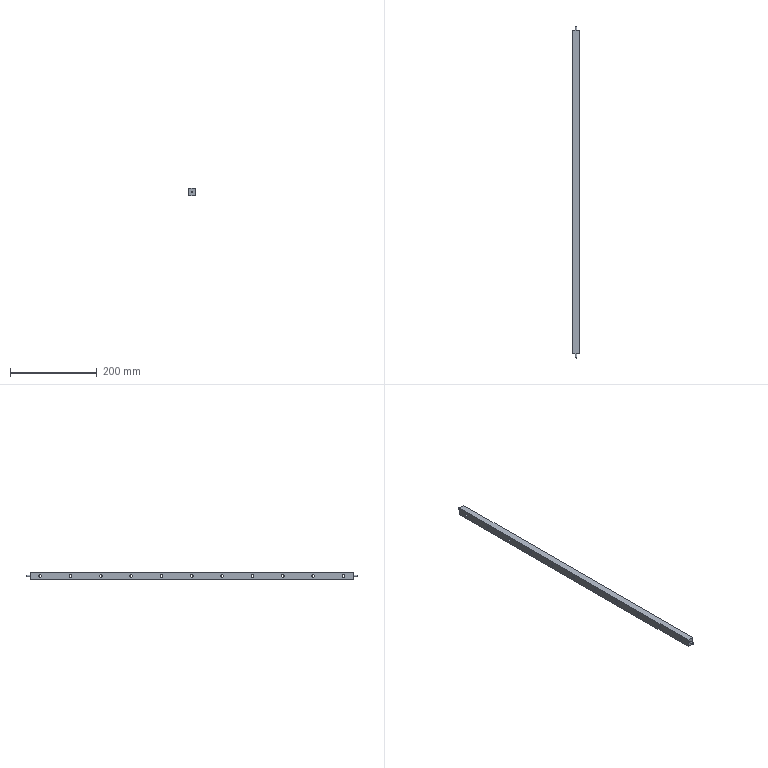Component | NX | CROSS_BAR_4 | 1 solid | 21 faces | volume 196186 mm3 | cylinder 13 | plane 8 | commonest cylinder face diameters 6 x11 4 x2